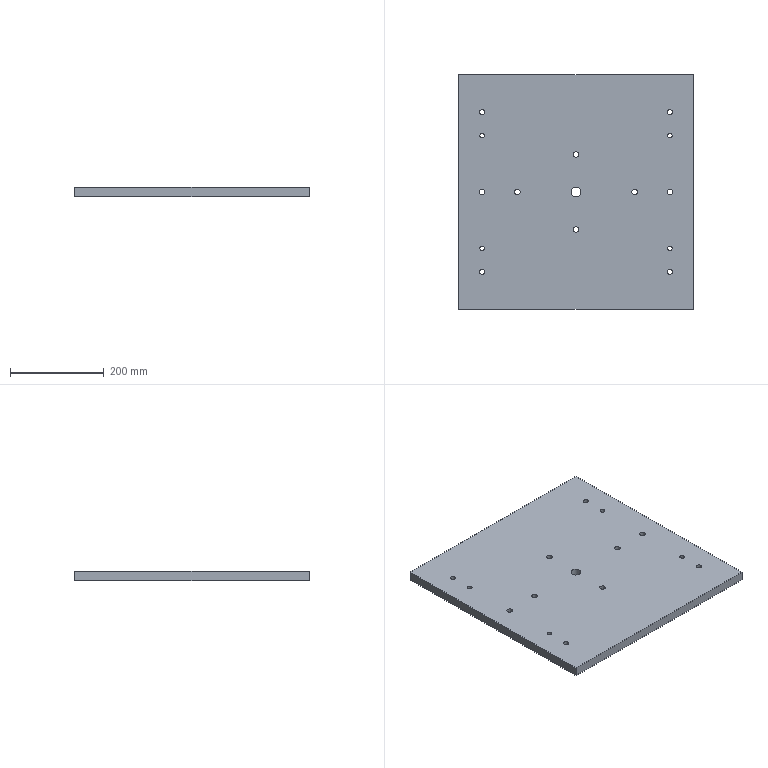Component | NX | SPACER_PLATE | 1 solid | 21 faces | volume 4965615 mm3 | cylinder 15 | plane 6 | commonest cylinder face diameters 12 x6 10 x4 11 x4 21 x1